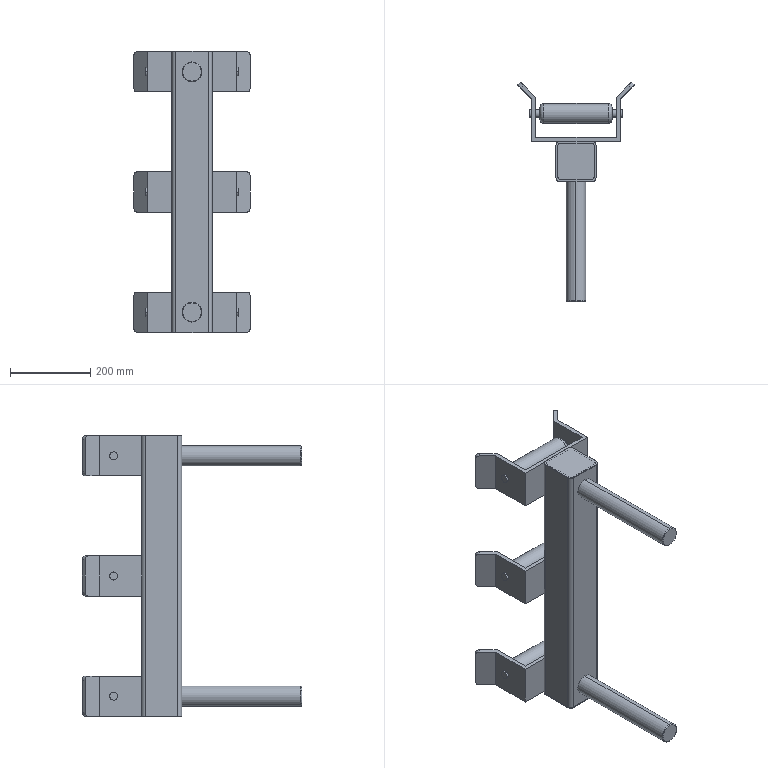Component | SolidWorks | IdlerRoller-1 | 17 solids | 164 faces | box 290.71 x 548.28 x 704 mm | volume 5129817 mm3 | plane 86 | cylinder 62 | torus 14 | cone 2 | commonest cylinder face diameters 20 x48 50 x10 10 x4 | material 45
build123d program:
from build123d import *

# Parameters (mm, degrees)
BOSS_EXTRUDE1_DEPTH      = 100
BOSS_EXTRUDE2_DEPTH      = 90
BOSS_EXTRUDE2_DEPTH_BACK = 90
SKETCH2_2_R              = 25
FILLET1_R                = 10
FILLET2_R                = 10
SKETCH1_R                = 10
CUT_EXTRUDE1_DEPTH       = 15
CUT_EXTRUDE2_START       = -15
SKETCH2_R                = 10
CUT_EXTRUDE2_DEPTH       = 15
SKETCH3_R                = 10
BOSS_EXTRUDE3_DEPTH      = 25
LPATTERN1_COUNT          = 3
LPATTERN1_PITCH          = 300
BOSS_EXTRUDE4_DEPTH      = 700
BOSS_EXTRUDE5_DEPTH      = 2
BOSS_EXTRUDE6_DEPTH      = 2
SKETCH7_R                = 25
BOSS_EXTRUDE7_DEPTH      = 300
BOSS_EXTRUDE7_2_DEPTH    = 300
CHAMFER1_SIZE            = 2
FILLET3_R                = 2


with BuildPart() as part:
    # Sketch1_2 → Boss-Extrude1 (new body)
    with BuildSketch(Plane.XY):
        Polygon((0, 0), (35.355, -35.355), (35.355, -141.213), (255.355, -141.213), (255.355, -35.355), (290.711, 0), (283.64, 7.071), (245.355, -31.213), (245.355, -131.213), (45.355, -131.213), (45.355, -31.213), (7.071, 7.071), align=None)
    extrude(amount=BOSS_EXTRUDE1_DEPTH)

    # Fillet2
    fillet2_edges = [part.edges().sort_by_distance(p)[0] for p in [
        (287.175, 3.536, 0),
        (3.536, 3.536, 0),
        (287.175, 3.536, 100),
        (3.536, 3.536, 100),
    ]]
    fillet(fillet2_edges, radius=FILLET2_R)

    # Sketch1 → Cut-Extrude1 (cut)
    with BuildSketch(Plane.ZY.offset(-35.355)):
        with Locations((50, -71.213)):
            Circle(SKETCH1_R)
    extrude(amount=-CUT_EXTRUDE1_DEPTH, mode=Mode.SUBTRACT)

    # Sketch2 → Cut-Extrude2 (cut)
    with BuildSketch(Plane(origin=(255.355, 0, 0), x_dir=(0, 0, -1), z_dir=(1, 0, 0)).offset(CUT_EXTRUDE2_START)):
        with Locations(Location((-50, -71.213, 0), (0, 0, 180))):
            Circle(SKETCH2_R)
    extrude(amount=CUT_EXTRUDE2_DEPTH, mode=Mode.SUBTRACT)


with BuildPart() as body_2:
    # Sketch2_2 → Boss-Extrude2 (new, two sides: drawn at the far end of the back side and taken through both)
    with BuildSketch(Plane.ZY.offset(-145.355).offset(-BOSS_EXTRUDE2_DEPTH_BACK)):
        with Locations(Location((50, -71.213, 0), (0, 0, 90))):
            Circle(SKETCH2_2_R)
    extrude(amount=BOSS_EXTRUDE2_DEPTH + BOSS_EXTRUDE2_DEPTH_BACK)

    # Fillet1
    fillet1_edges = [body_2.edges().sort_by_distance(p)[0] for p in [
        (235.355, -96.213, 50),
        (55.355, -96.213, 50),
    ]]
    fillet(fillet1_edges, radius=FILLET1_R)


with BuildPart() as body_3:
    # Sketch3 → Boss-Extrude3 (new body)
    with BuildSketch(Plane.ZY.offset(-55.355)):
        with Locations(Location((50, -71.213, 0), (0, 0, 90))):
            Circle(SKETCH3_R)
    extrude(amount=BOSS_EXTRUDE3_DEPTH)


with BuildPart() as body_4:
    # Mirror2: mirrored copy
    add(body_3.part.mirror(Plane.ZY.offset(-145.355)))


with BuildPart() as lpattern1_1:
    # LPattern1: pattern copy
    add(body_3.part.moved(Location(Vector(0, 0, -1) * (1 * LPATTERN1_PITCH))))


with BuildPart() as lpattern1_2:
    # LPattern1: pattern copy
    add(body_3.part.moved(Location(Vector(0, 0, -1) * (2 * LPATTERN1_PITCH))))


with BuildPart() as lpattern1_3:
    # LPattern1: pattern copy
    add(part.part.moved(Location(Vector(0, 0, -1) * (1 * LPATTERN1_PITCH))))


with BuildPart() as lpattern1_4:
    # LPattern1: pattern copy
    add(part.part.moved(Location(Vector(0, 0, -1) * (2 * LPATTERN1_PITCH))))


with BuildPart() as lpattern1_5:
    # LPattern1: pattern copy
    add(body_2.part.moved(Location(Vector(0, 0, -1) * (1 * LPATTERN1_PITCH))))


with BuildPart() as lpattern1_6:
    # LPattern1: pattern copy
    add(body_2.part.moved(Location(Vector(0, 0, -1) * (2 * LPATTERN1_PITCH))))


with BuildPart() as lpattern1_7:
    # LPattern1: pattern copy
    add(body_4.part.moved(Location(Vector(0, 0, -1) * (1 * LPATTERN1_PITCH))))


with BuildPart() as lpattern1_8:
    # LPattern1: pattern copy
    add(body_4.part.moved(Location(Vector(0, 0, -1) * (2 * LPATTERN1_PITCH))))


with BuildPart() as body_13:
    # Sketch4 → Boss-Extrude4 (new body)
    with BuildSketch(Plane.XY.offset(100)):
        with BuildLine():
            Line((185.355, -241.213), (105.355, -241.213))
            ThreePointArc((105.355, -241.213), (98.284, -238.284), (95.355, -231.213))
            Line((95.355, -231.213), (95.355, -151.213))
            ThreePointArc((95.355, -151.213), (98.284, -144.142), (105.355, -141.213))
            Line((105.355, -141.213), (185.355, -141.213))
            ThreePointArc((185.355, -141.213), (192.426, -144.142), (195.355, -151.213))
            Line((195.355, -151.213), (195.355, -231.213))
            ThreePointArc((195.355, -231.213), (192.426, -238.284), (185.355, -241.213))
        make_face()
        with BuildLine():
            Line((100.355, -231.213), (100.355, -151.213))
            ThreePointArc((100.355, -151.213), (101.82, -147.678), (105.355, -146.213))
            Line((105.355, -146.213), (185.355, -146.213))
            ThreePointArc((185.355, -146.213), (188.891, -147.678), (190.355, -151.213))
            Line((190.355, -151.213), (190.355, -231.213))
            ThreePointArc((190.355, -231.213), (188.891, -234.749), (185.355, -236.213))
            Line((185.355, -236.213), (105.355, -236.213))
            ThreePointArc((105.355, -236.213), (101.82, -234.749), (100.355, -231.213))
        make_face(mode=Mode.SUBTRACT)
    extrude(amount=-BOSS_EXTRUDE4_DEPTH)


with BuildPart() as body_14:
    # Sketch5 → Boss-Extrude5 (new body)
    with BuildSketch(Plane.XY.offset(100)):
        with BuildLine():
            Line((195.355, -231.213), (195.355, -151.213))
            ThreePointArc((195.355, -151.213), (192.426, -144.142), (185.355, -141.213))
            Line((185.355, -141.213), (105.355, -141.213))
            ThreePointArc((105.355, -141.213), (98.284, -144.142), (95.355, -151.213))
            Line((95.355, -151.213), (95.355, -231.213))
            ThreePointArc((95.355, -231.213), (98.284, -238.284), (105.355, -241.213))
            Line((105.355, -241.213), (185.355, -241.213))
            ThreePointArc((185.355, -241.213), (192.426, -238.284), (195.355, -231.213))
        make_face()
    extrude(amount=BOSS_EXTRUDE5_DEPTH)


with BuildPart() as body_15:
    # Sketch6 → Boss-Extrude6 (new body)
    with BuildSketch(Plane(origin=(0, 0, -600), x_dir=(-1, 0, 0), z_dir=(0, 0, -1))):
        with BuildLine():
            Line((-185.355, -241.213), (-105.355, -241.213))
            ThreePointArc((-105.355, -241.213), (-98.284, -238.284), (-95.355, -231.213))
            Line((-95.355, -231.213), (-95.355, -151.213))
            ThreePointArc((-95.355, -151.213), (-98.284, -144.142), (-105.355, -141.213))
            Line((-105.355, -141.213), (-185.355, -141.213))
            ThreePointArc((-185.355, -141.213), (-192.426, -144.142), (-195.355, -151.213))
            Line((-195.355, -151.213), (-195.355, -231.213))
            ThreePointArc((-195.355, -231.213), (-192.426, -238.284), (-185.355, -241.213))
        make_face()
    extrude(amount=BOSS_EXTRUDE6_DEPTH)


with BuildPart() as body_16:
    # Sketch7 → Boss-Extrude7 (new body)
    with BuildSketch(Plane.XZ.offset(241.213)):
        with Locations(Location((145.355, 50, 0), (0, 0, 270))):
            Circle(SKETCH7_R)
    extrude(amount=BOSS_EXTRUDE7_DEPTH)

    # Chamfer1
    chamfer1_edges = [body_16.edges().sort_by_distance(p)[0] for p in [
        (145.355, -541.213, 75),
    ]]
    chamfer(chamfer1_edges, length=CHAMFER1_SIZE)


with BuildPart() as body_17:
    # Sketch7 → Boss-Extrude7 2 (new body)
    with BuildSketch(Plane.XZ.offset(241.213)):
        with Locations(Location((145.355, -550, 0), (0, 0, 270))):
            Circle(SKETCH7_R)
    extrude(amount=BOSS_EXTRUDE7_2_DEPTH)

    # Fillet3
    fillet3_edges = [body_17.edges().sort_by_distance(p)[0] for p in [
        (145.355, -541.213, -525),
    ]]
    fillet(fillet3_edges, radius=FILLET3_R)


solid = Compound([part.part, body_2.part, body_3.part, body_4.part, lpattern1_1.part, lpattern1_2.part, lpattern1_3.part, lpattern1_4.part, lpattern1_5.part, lpattern1_6.part, lpattern1_7.part, lpattern1_8.part, body_13.part, body_14.part, body_15.part, body_16.part, body_17.part])

# Placed as in the assembly
solid = solid.moved(Location((-236.168, 229.642, 350), (0, 0, 0)))